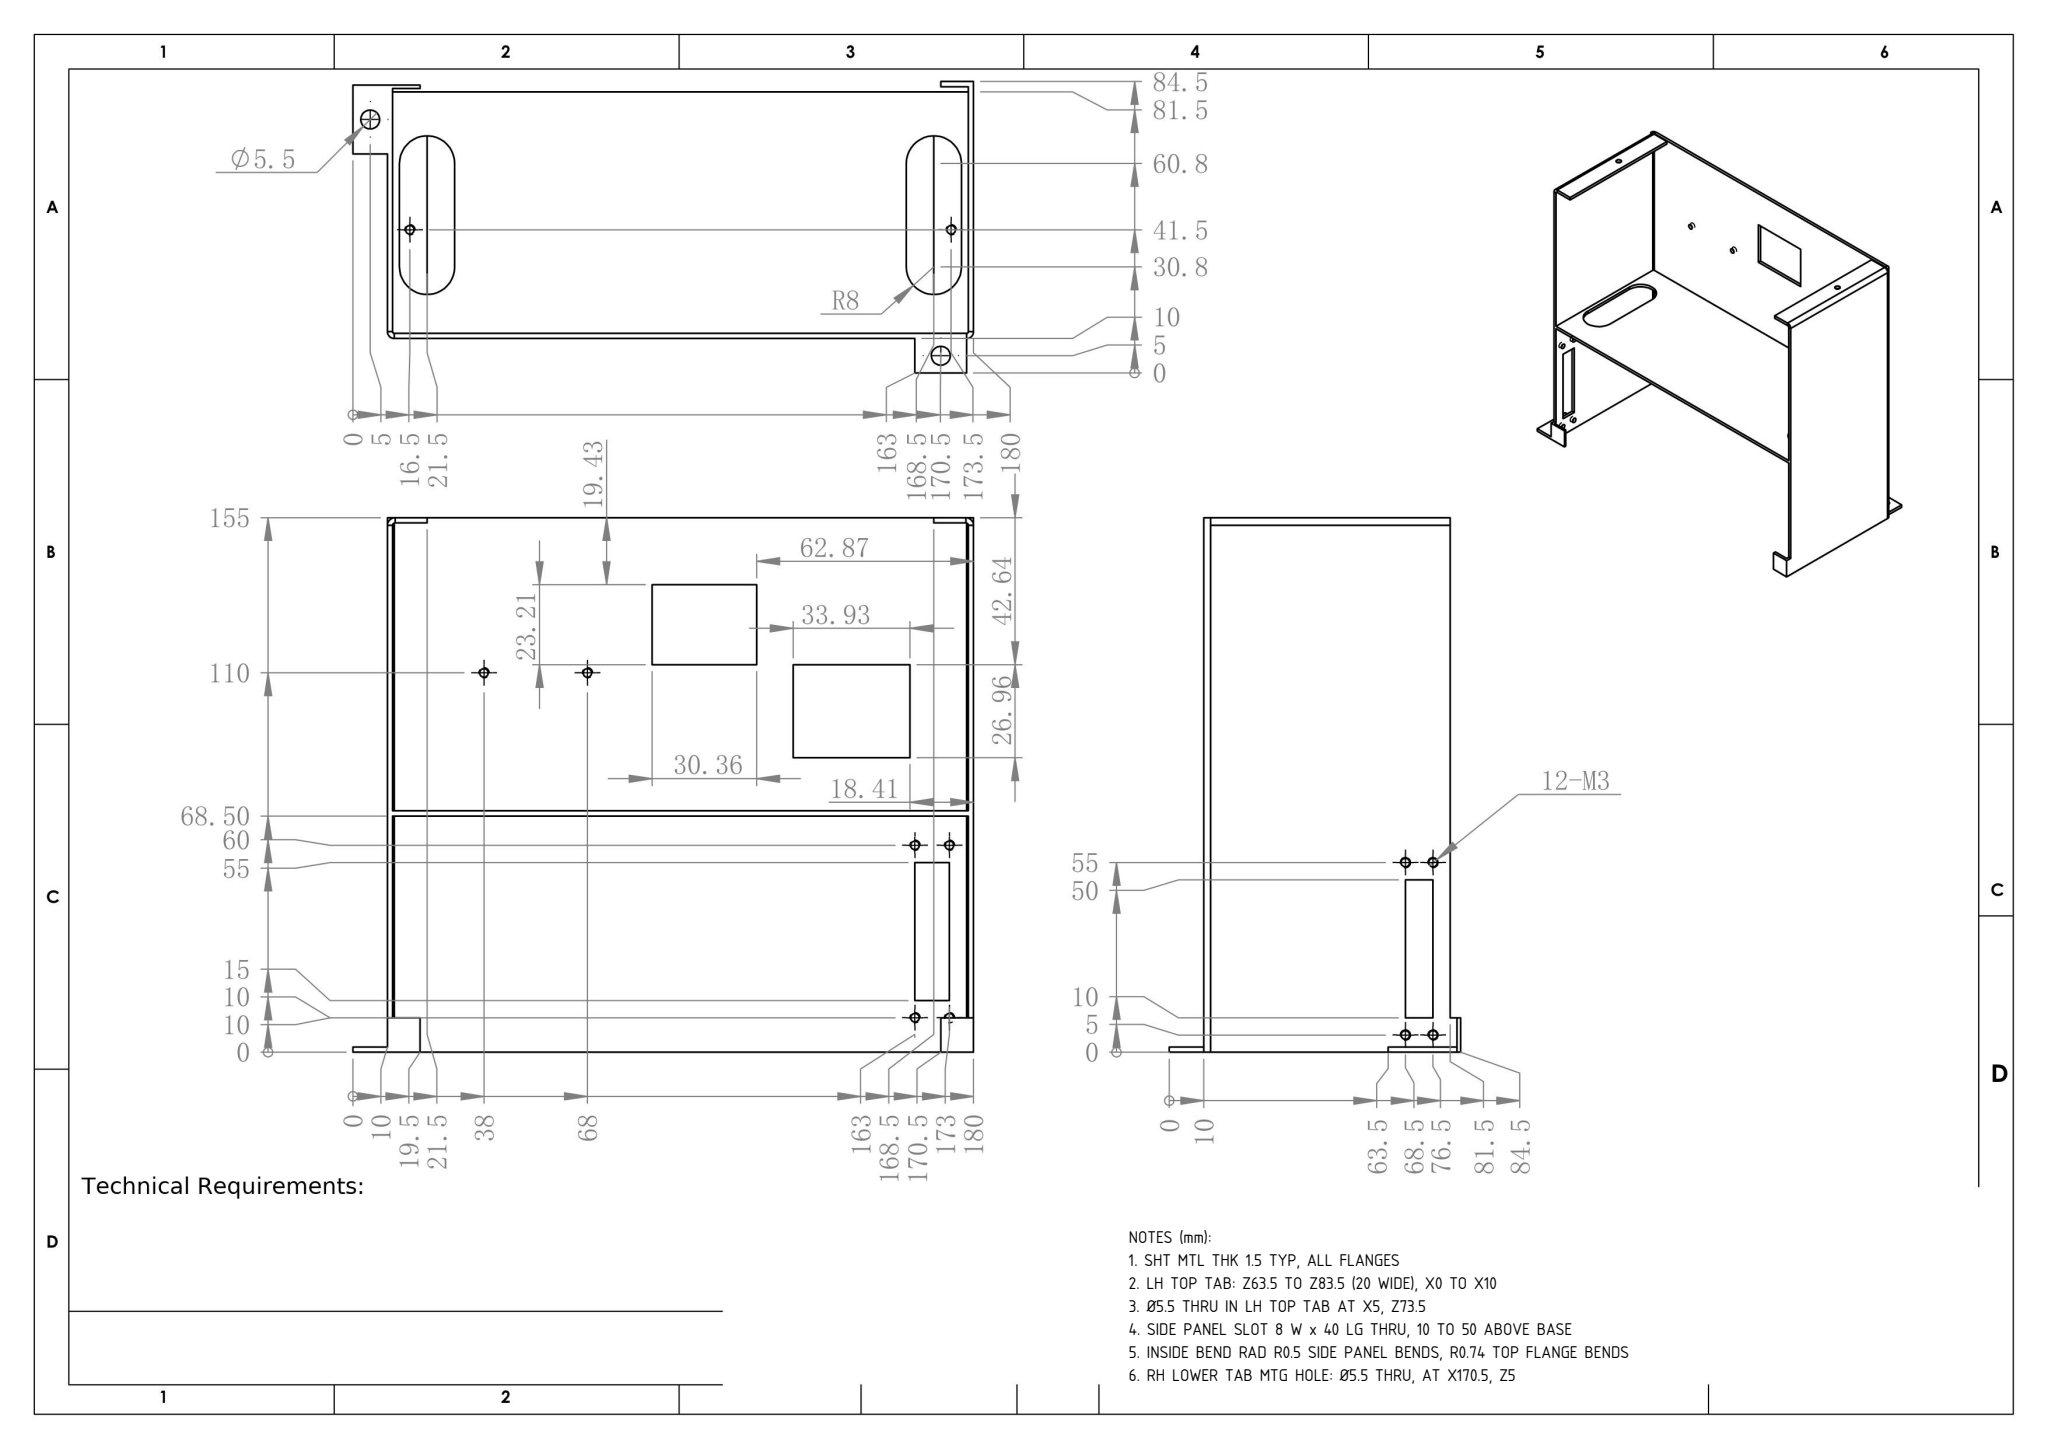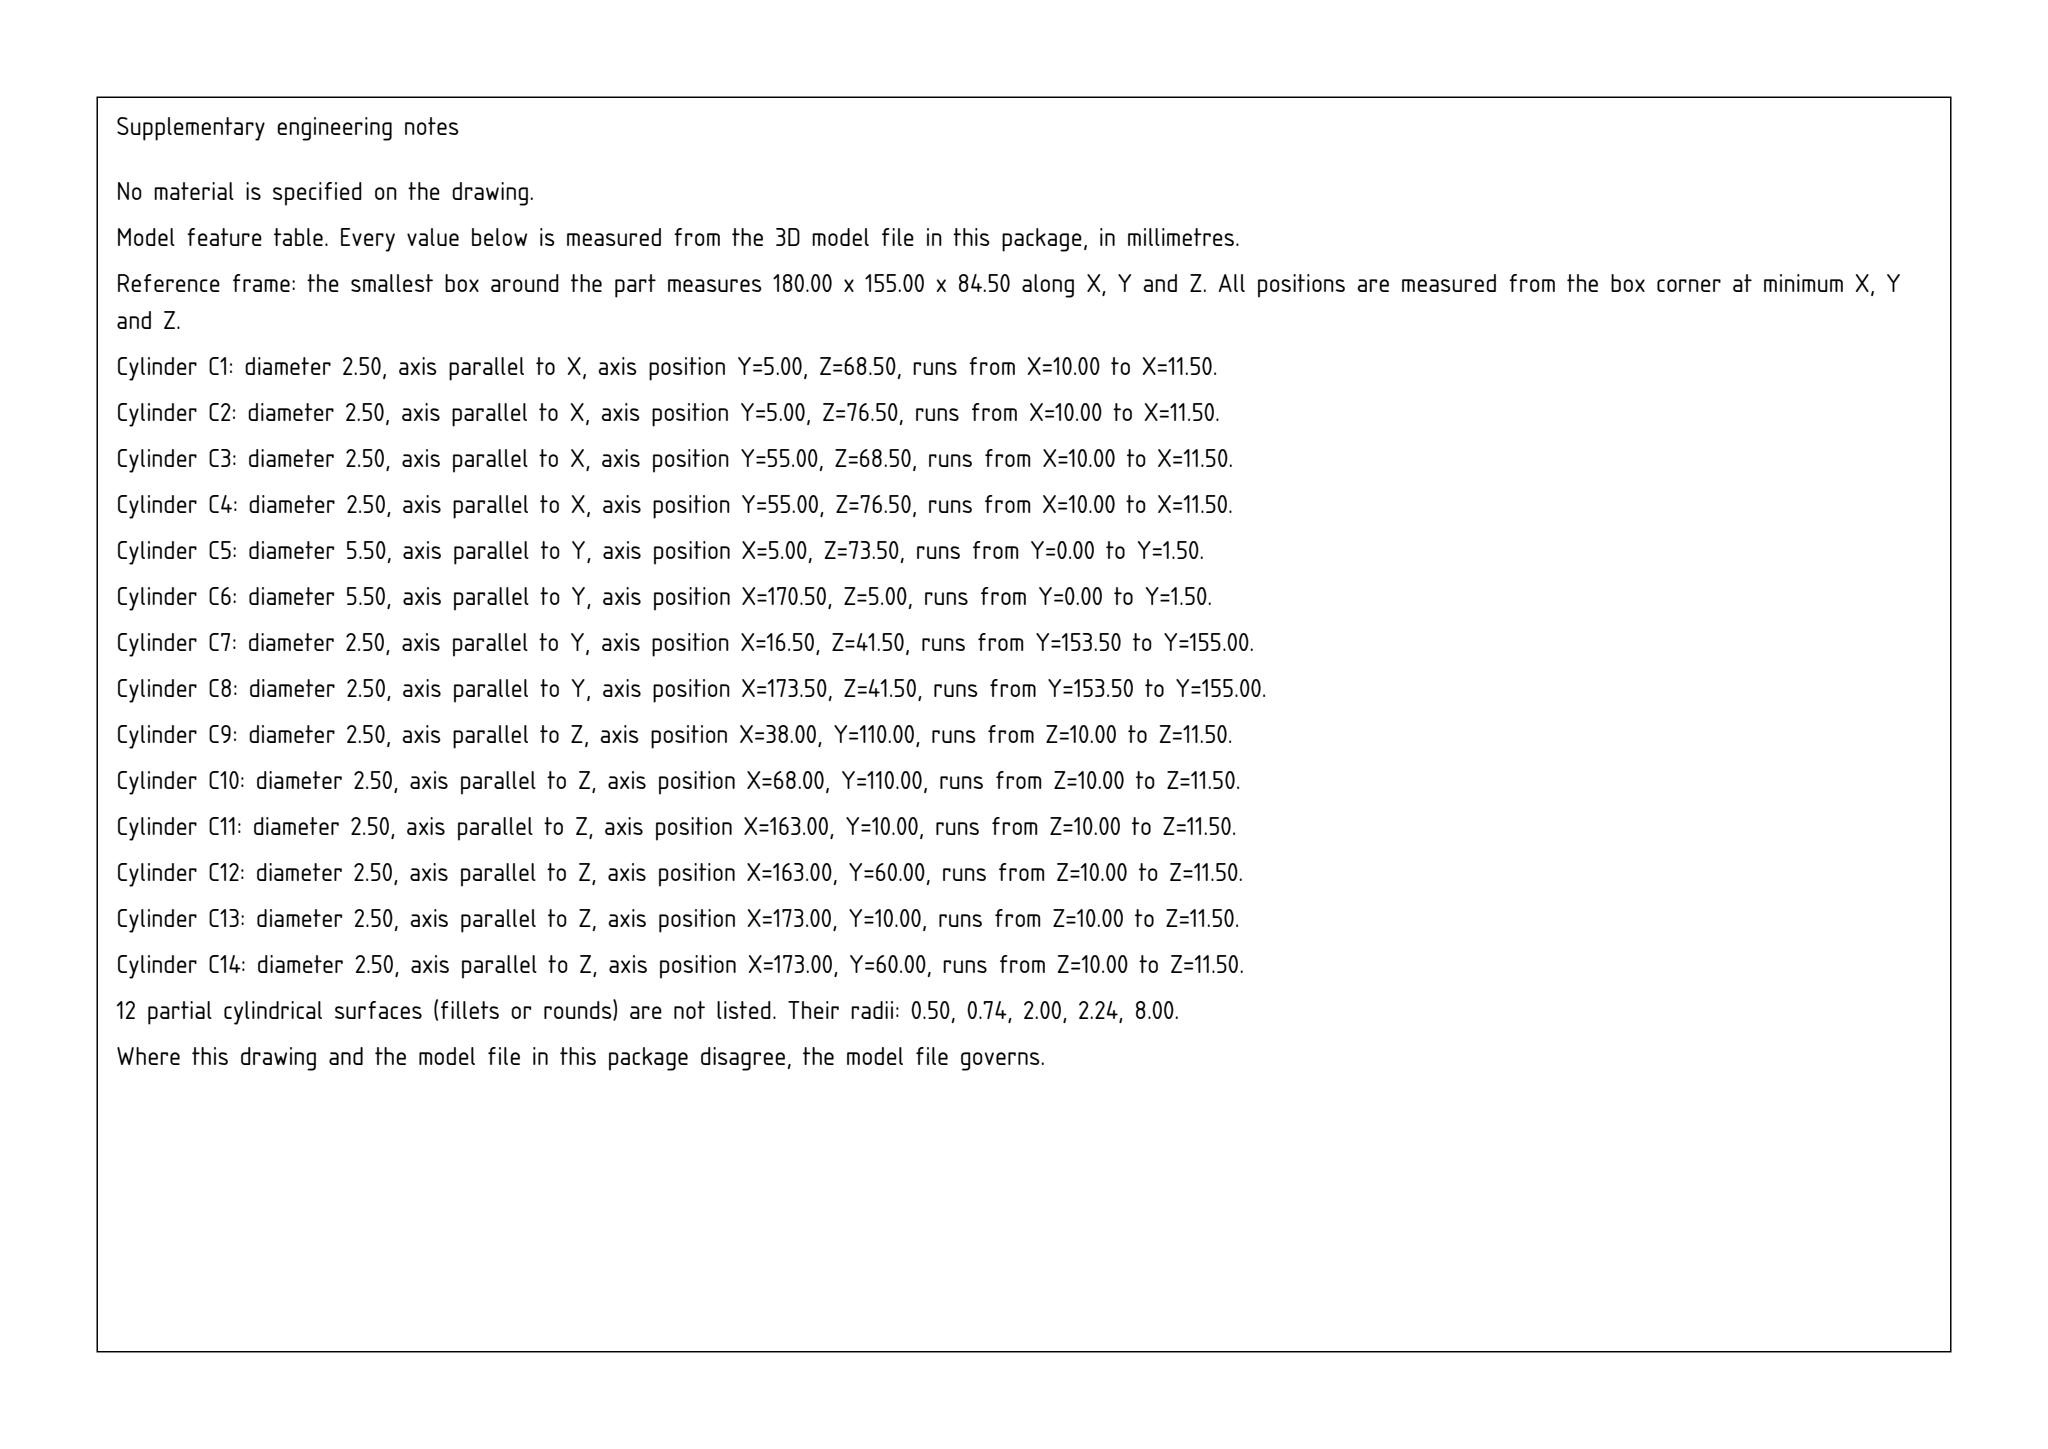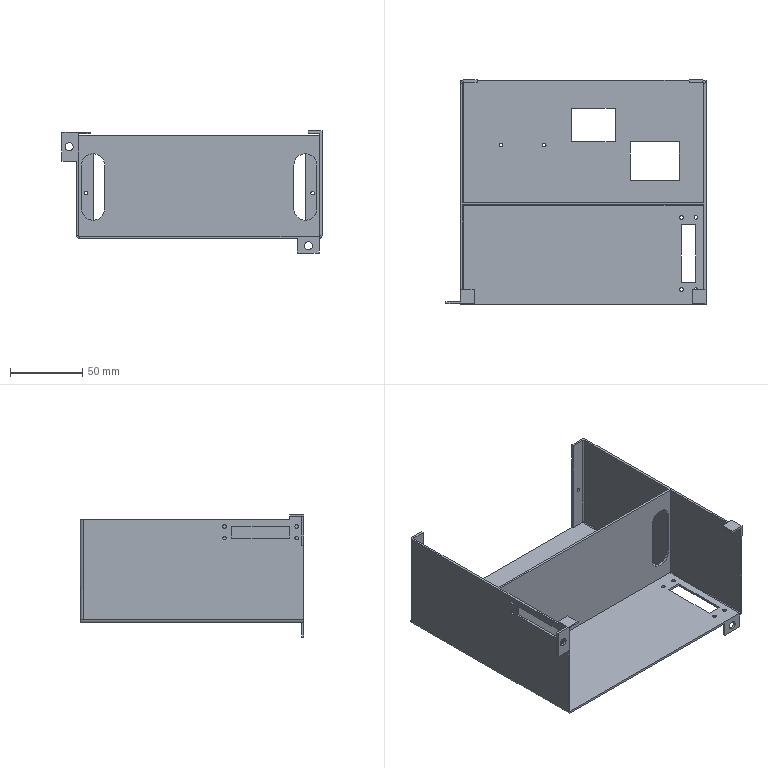Part | SolidWorks | mm | 1 solid | 115 faces | box 180 x 155 x 84.5 mm | volume 86400 mm3 | plane 71 | cylinder 44 | commonest cylinder face diameters 2.5 x24 16 x6 5.5 x4 1 x4 4 x2 4.473 x2 1.473 x2
Drawing notes:
SHT MTL THK 1.5 TYP, ALL FLANGES | from the solid: All thru features len 1.5; paired planes x10.0/11.5, z11.5/12.0, x178.5/180.0 give 1.5 wall
LH TOP TAB: Z63.5 TO Z83.5 (20 WIDE), X0 TO X10 | from the solid: axis planes z=63.5 and z=83.5, x=0 and x=10.0 bound the upper-left mounting tab
Ø5.5 THRU IN LH TOP TAB AT X5, Z73.5 | from the solid: cylinder [5.5,"y",[5.0,null,73.5],1.5] -> X=5, Z=73.5 from bbox min corner (drawing Z0 datum)
SIDE PANEL SLOT 8 W x 40 LG THRU, 10 TO 50 ABOVE BASE | from the solid: z planes 68.5/76.5 (8 wide) with y planes 10/50 (40 long) in 1.5 thk side wall
INSIDE BEND RAD R0.5 SIDE PANEL BENDS, R0.74 TOP FLANGE BENDS | from the solid: STEP inner bend radii ~R0.5 at vertical side-panel bends, ~R0.74 at top flange bends
RH LOWER TAB MTG HOLE: Ø5.5 THRU, AT X170.5, Z5 | from the solid: cylinder dia 5.5, axis y, pos (170.5, -, 5.0), length 1.5 (tab thk)